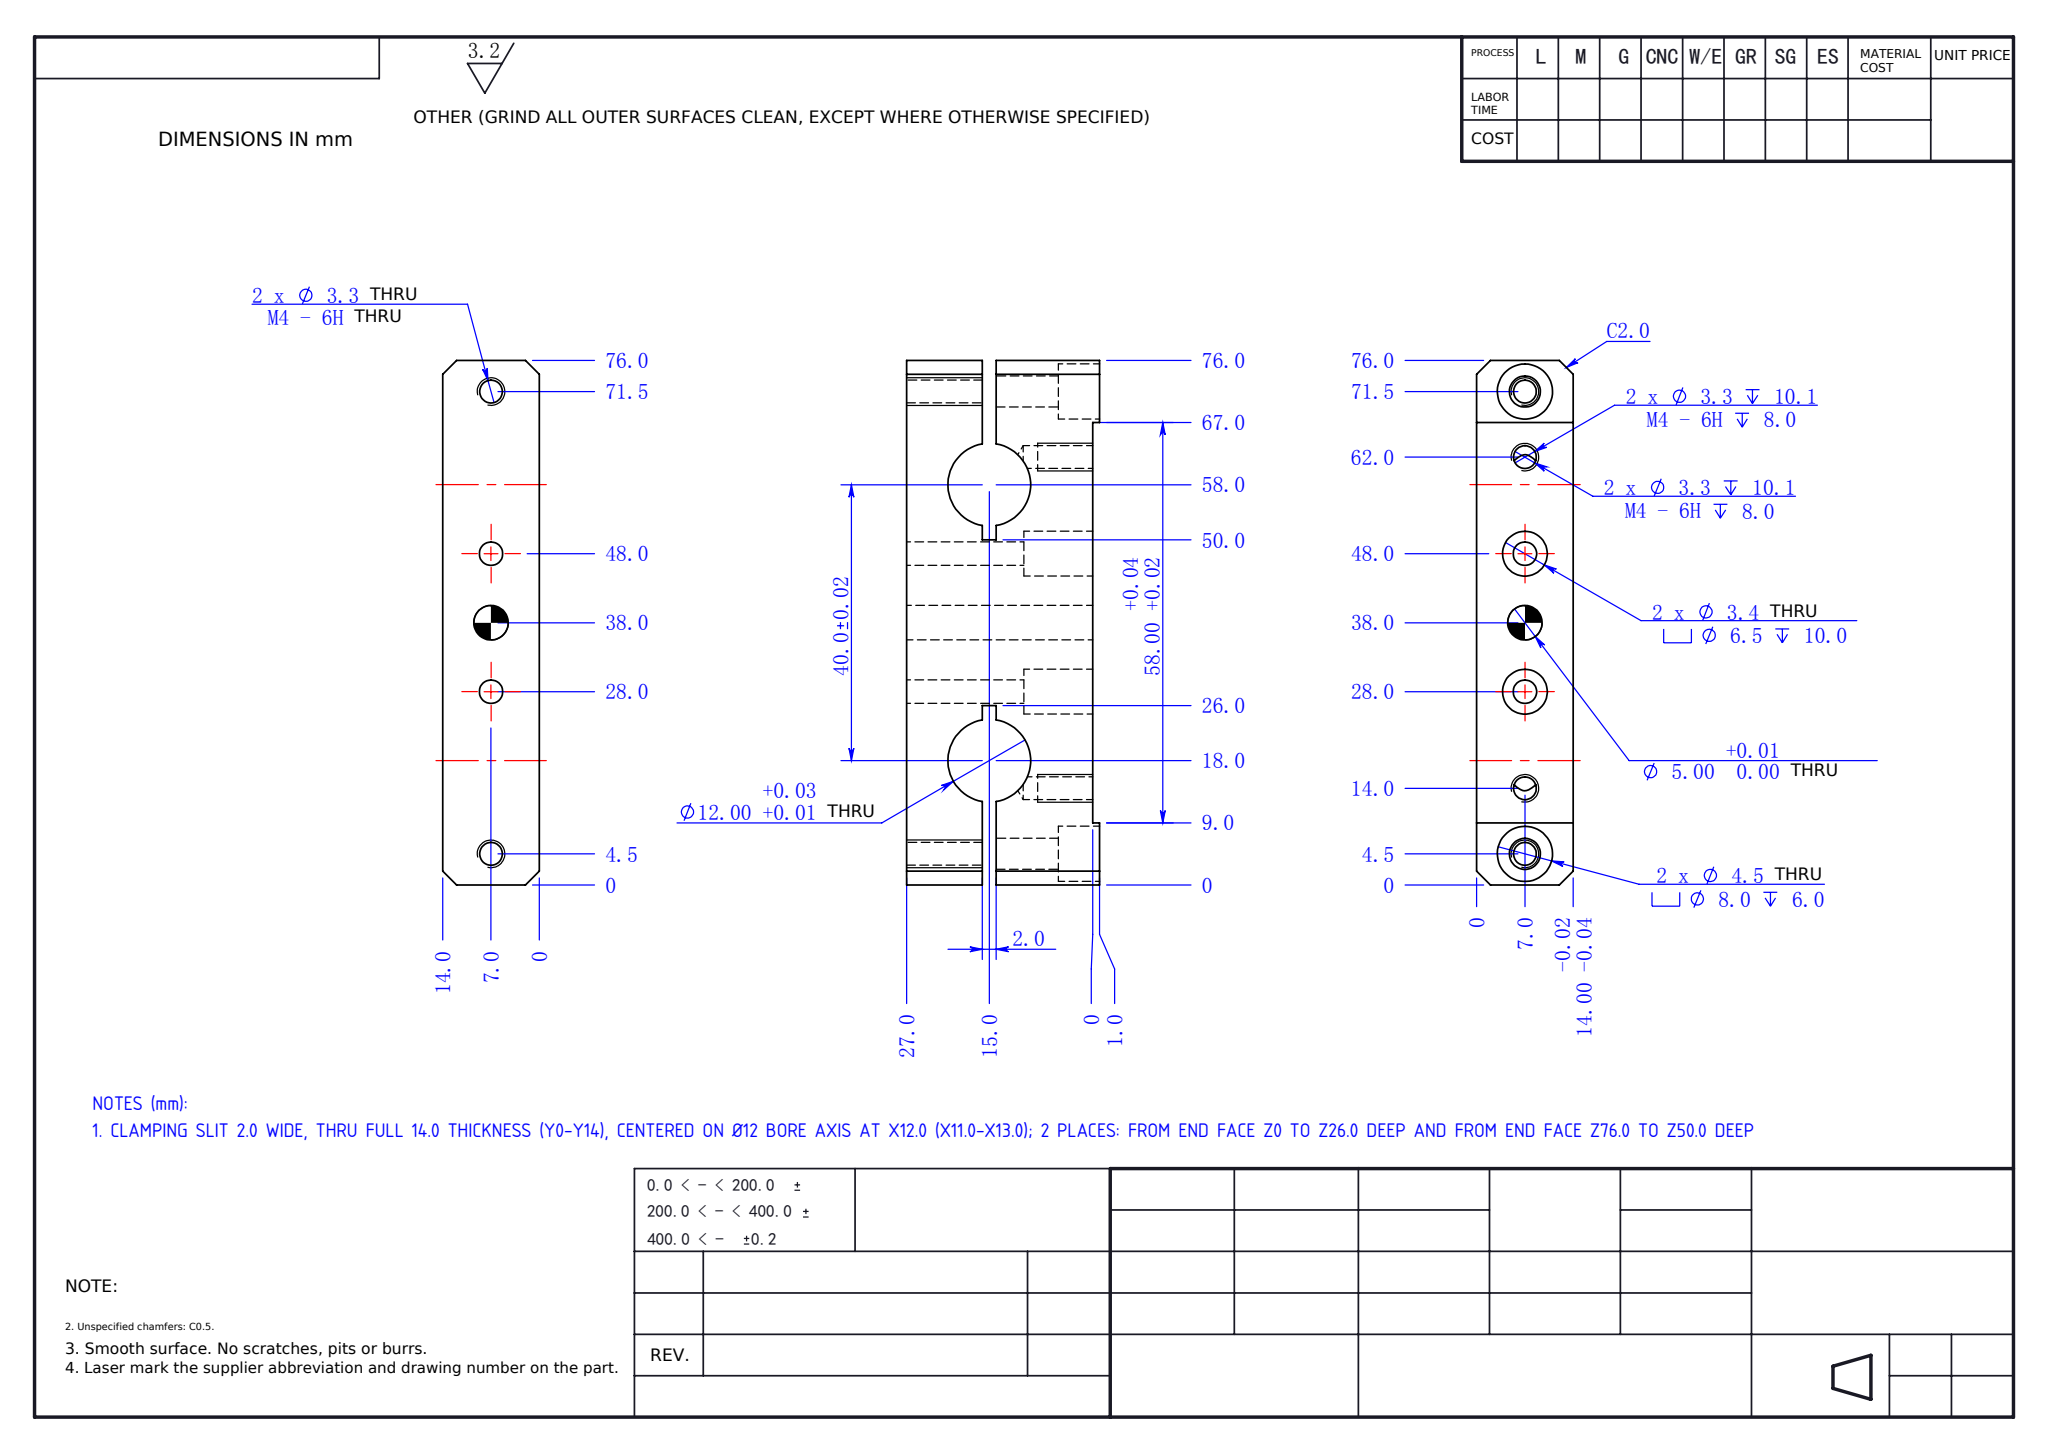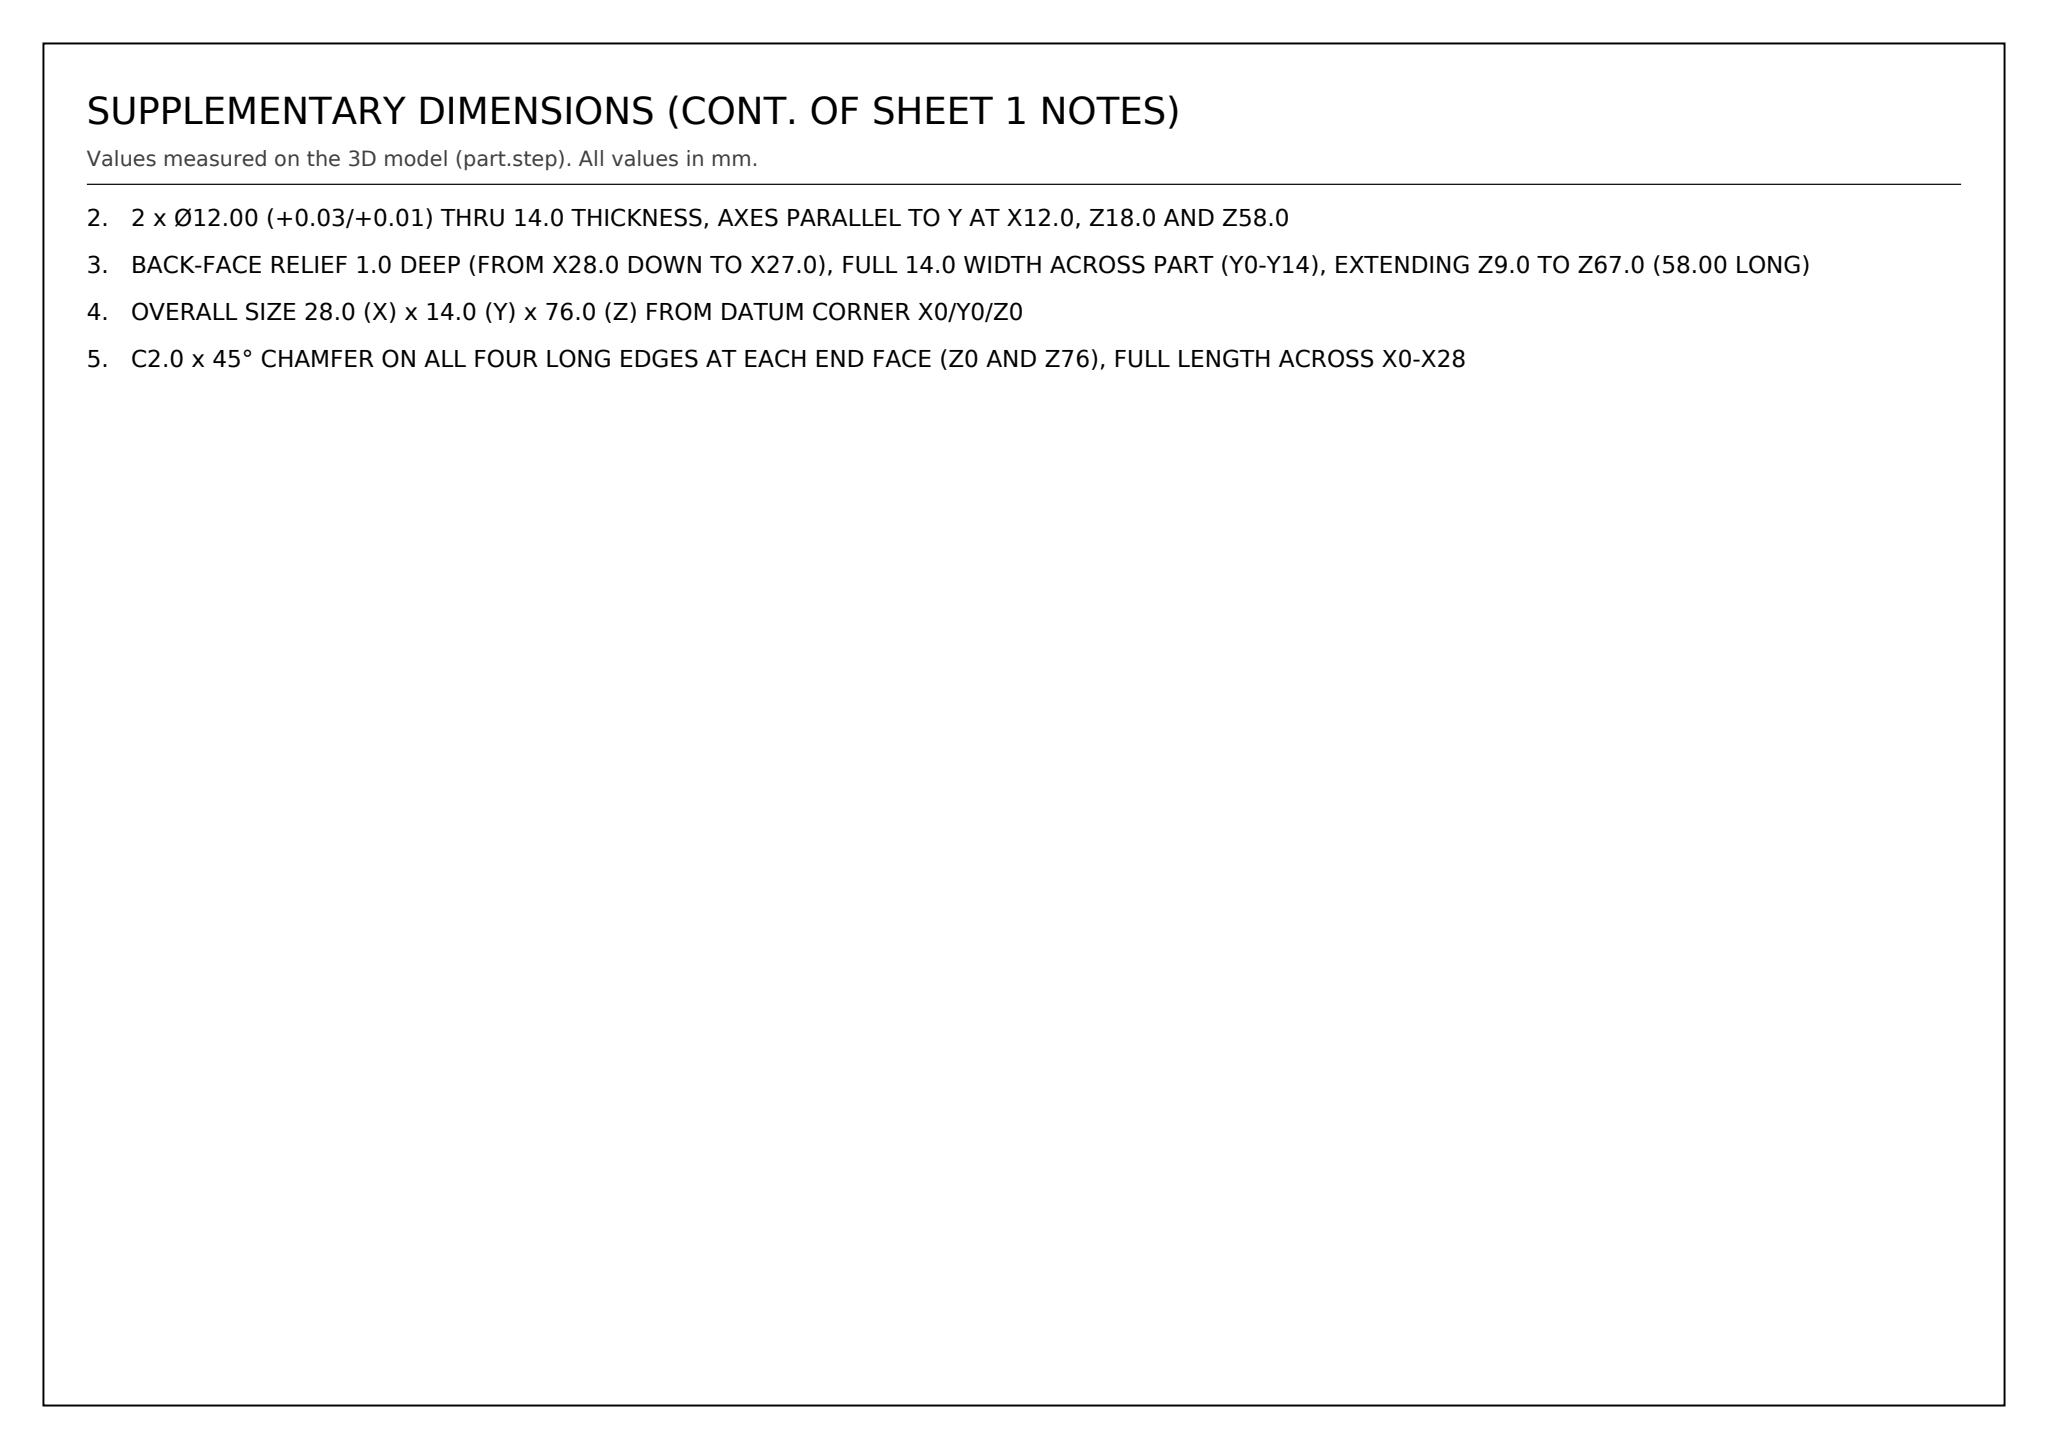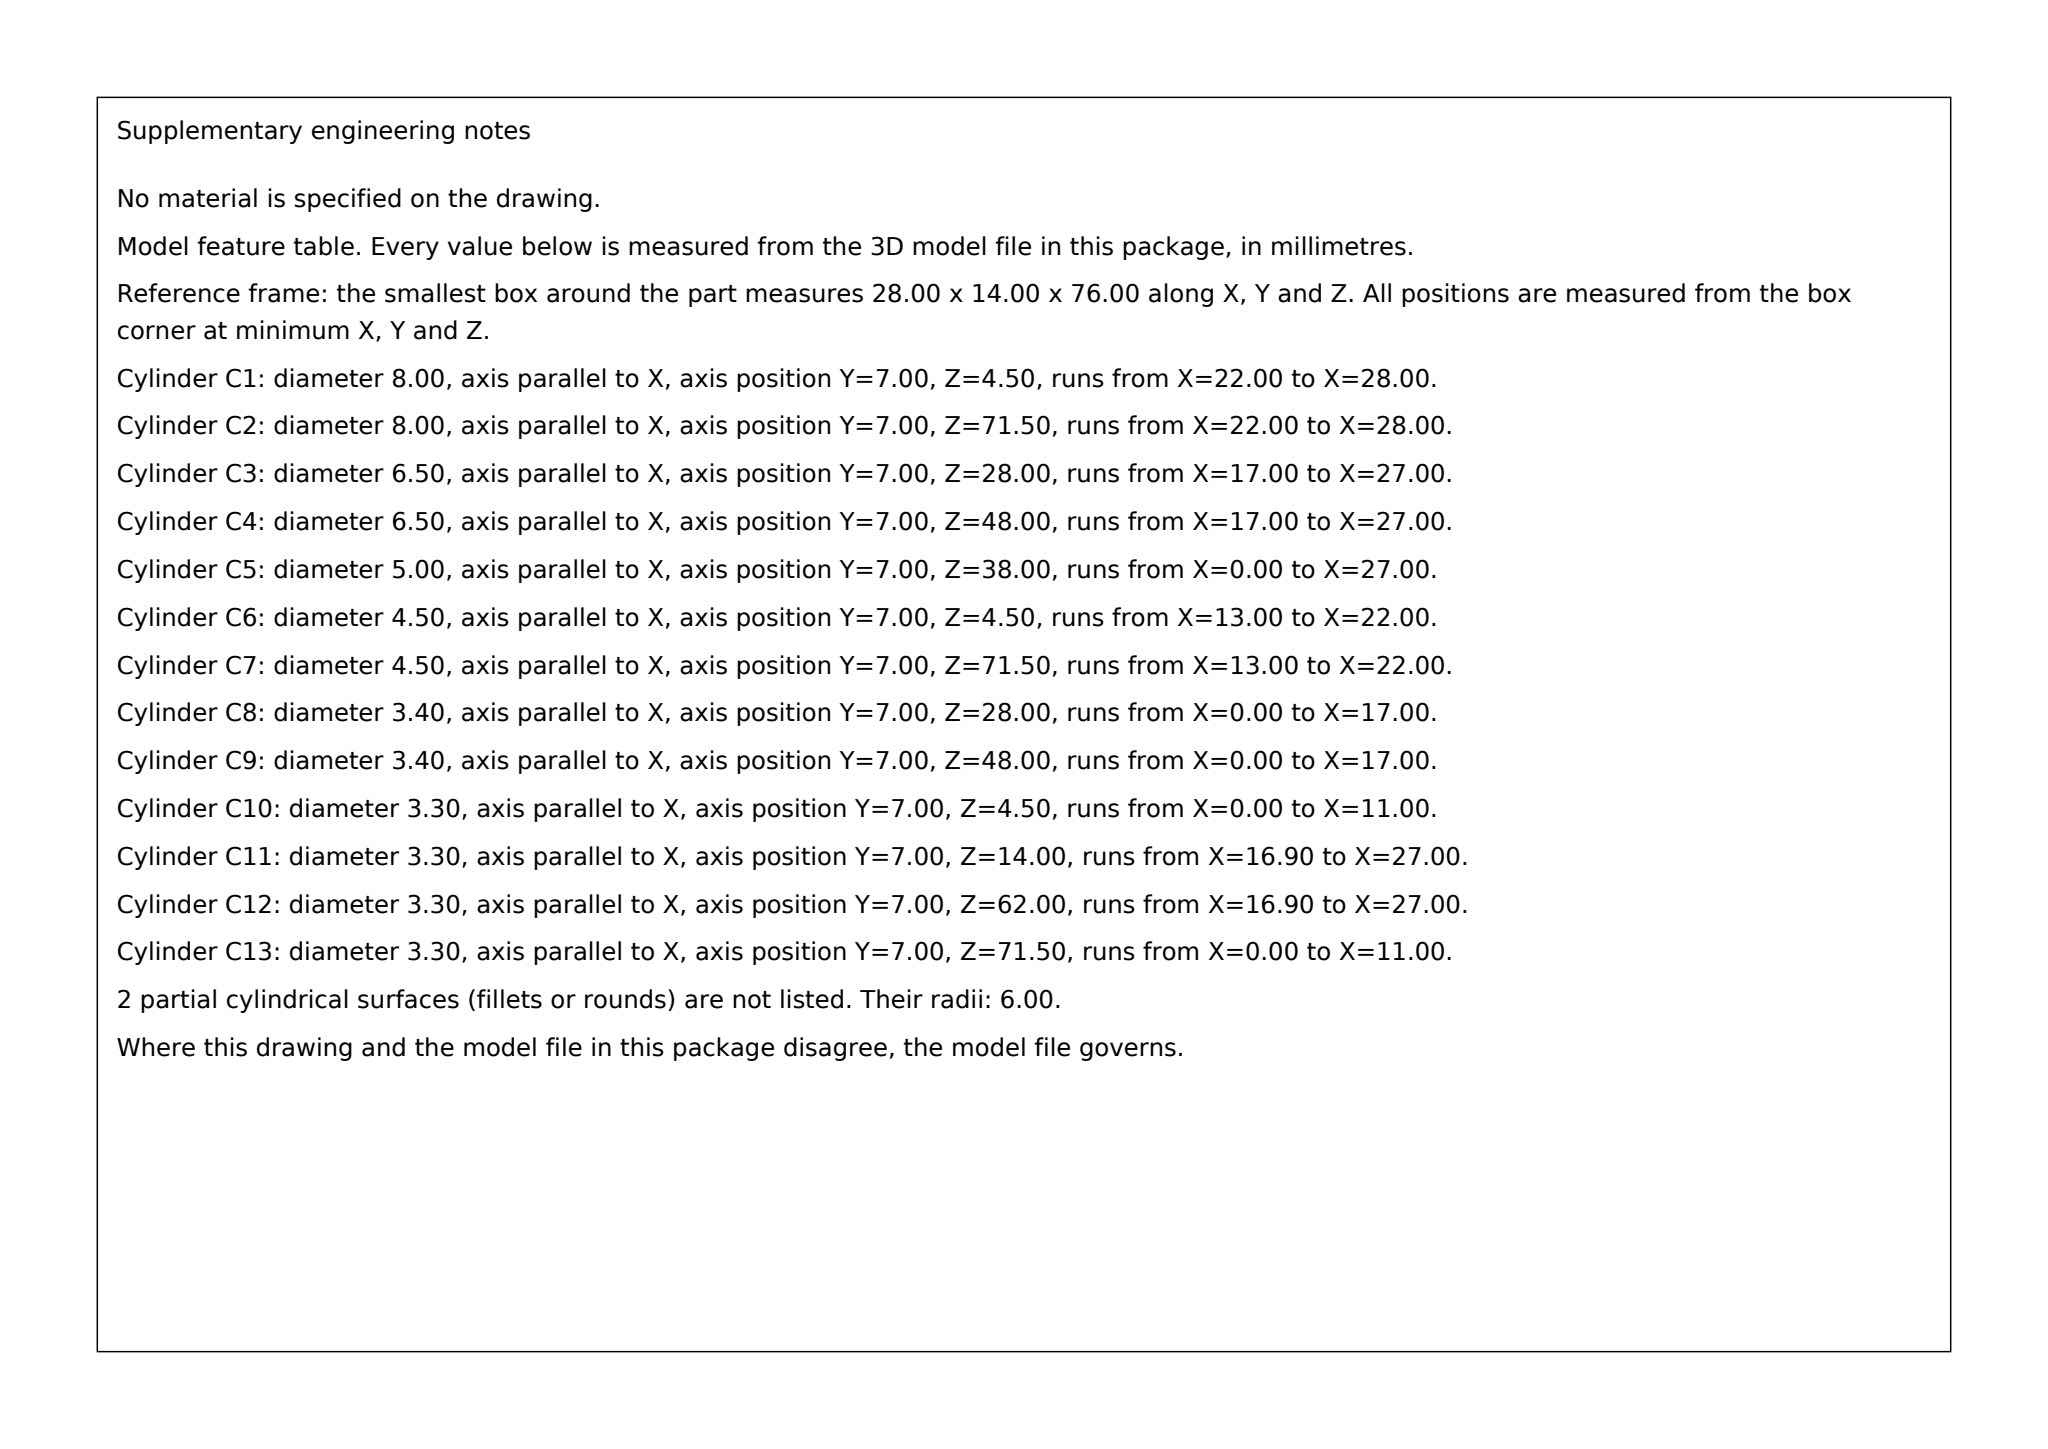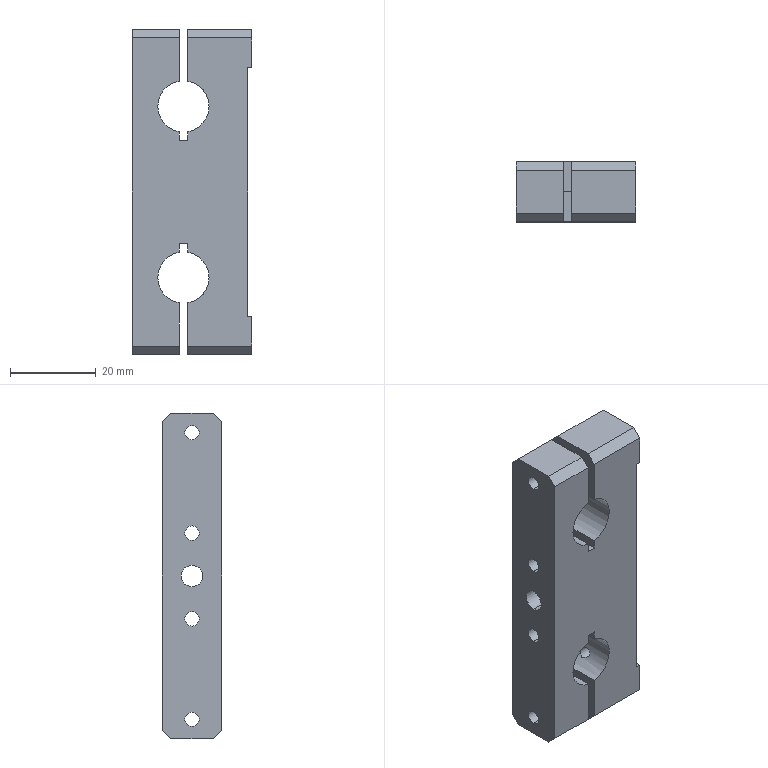Part | SolidWorks | mm | 1 solid | 67 faces | box 28 x 14 x 76 mm | volume 22063 mm3 | plane 34 | cylinder 30 | cone 3 | commonest cylinder face diameters 3.3 x8 8 x4 4.5 x4 6.5 x4 3.4 x4 12 x4 5 x2
Drawing notes:
CLAMPING SLIT 2.0 WIDE, THRU FULL 14.0 THICKNESS (Y0-Y14), CENTERED ON Ø12 BORE AXIS AT X12.0 (X11.0-X13.0); 2 PLACES: FROM END FACE Z0 TO Z26.0 DEEP AND FROM END FACE Z76.0 TO Z50.0 DEEP | from the solid: axis_planes x=11.0 and x=13.0, y extent [0,14], z extents [0,12.1],[23.9,26.0],[50.0,52.1],[63.9,76.0]; end planes z=26.0 and z=50.0 over x [11,13]
2 x Ø12.00 (+0.03/+0.01) THRU 14.0 THICKNESS, AXES PARALLEL TO Y AT X12.0, Z18.0 AND Z58.0 | from the solid: cylinders: two 12.0 dia arcs, axis y, positions [12.0,-,18.0] and [12.0,-,58.0], from y0 to y14
BACK-FACE RELIEF 1.0 DEEP (FROM X28.0 DOWN TO X27.0), FULL 14.0 WIDTH ACROSS PART (Y0-Y14), EXTENDING Z9.0 TO Z67.0 (58.00 LONG) | from the solid: axis_planes x=27.0 extent y[0,14] z[9,67]; x=28.0 extents z[0,9] and z[67,76]; z=9.0 and z=67.0 planes over x[27,28]
OVERALL SIZE 28.0 (X) x 14.0 (Y) x 76.0 (Z) FROM DATUM CORNER X0/Y0/Z0 | from the solid: bbox_xyz [28.0, 14.0, 76.0]
C2.0 x 45° CHAMFER ON ALL FOUR LONG EDGES AT EACH END FACE (Z0 AND Z76), FULL LENGTH ACROSS X0-X28 | from the solid: inclined_planes: eight 45° faces, size [11.0 or 15.0, 2.0, 2.0] at z=0 and z=74 origins, y=0 and y=12
build123d program:
from build123d import *

# Parameters (mm, degrees)
SKETCH1_W                                       = 28
SKETCH1_H                                       = 70
BOSS_EXTRUDE1_DEPTH                             = 7
SKETCH2_R                                       = 6
CUT_EXTRUDE1_DEPTH                              = 41.212
SKETCH3_W                                       = 2
SKETCH3_H                                       = 23
CUT_EXTRUDE2_DEPTH                              = 41.212
SKETCH8_W                                       = 1
SKETCH8_H                                       = 58
CUT_EXTRUDE5_DEPTH                              = 41.212
M4_TAPPED_HOLE2_D                               = 3.3
M4_TAPPED_HOLE2_DEPTH                           = 10.1
M4_TAPPED_HOLE2_TIP                             = 0.9914
M3_HEX_SOCKET_HEAD_CAP_SCREW_CBORE1_D           = 3.4
M3_HEX_SOCKET_HEAD_CAP_SCREW_CBORE1_CBORE_D     = 6.5
M3_HEX_SOCKET_HEAD_CAP_SCREW_CBORE1_CBORE_DEPTH = 10
SIZE_MM_DOWEL_PIN_HOLE_1_D                      = 5
SKETCH15_W                                      = 15
SKETCH15_H                                      = 14
SKETCH15_W_2                                    = 11
BOSS_EXTRUDE2_DEPTH                             = 3
SKETCH19_W                                      = 15
SKETCH19_H                                      = 14
SKETCH19_W_2                                    = 11
BOSS_EXTRUDE3_DEPTH                             = 3
M4_HEX_SOCKET_HEAD_CAP_SCREW_CBORE1_D           = 4.5
M4_HEX_SOCKET_HEAD_CAP_SCREW_CBORE1_DEPTH       = 15
M4_HEX_SOCKET_HEAD_CAP_SCREW_CBORE1_CBORE_D     = 8
M4_HEX_SOCKET_HEAD_CAP_SCREW_CBORE1_CBORE_DEPTH = 6
M4_TAPPED_HOLE3_D                               = 3.3
CHAMFER3_SIZE                                   = 2


with BuildPart() as part:
    # Sketch1 → Boss-Extrude1 (new, symmetric)
    with BuildSketch(Plane(origin=(0, 0, 0), x_dir=(1, 0, 0), z_dir=(0, 1, 0))):
        Rectangle(SKETCH1_W, SKETCH1_H)
    extrude(amount=BOSS_EXTRUDE1_DEPTH, both=True)

    # Sketch2 → Cut-Extrude1 (cut, through all)
    with BuildSketch(Plane(origin=(0, 7, 0), x_dir=(1, 0, 0), z_dir=(0, 1, 0))):
        with Locations(Location((-2, 20, 0), (0, 0, 270))):
            Circle(SKETCH2_R)
        with Locations(Location((-2, -20, 0), (0, 0, 90))):
            Circle(SKETCH2_R)
    extrude(amount=-CUT_EXTRUDE1_DEPTH, mode=Mode.SUBTRACT)

    # Sketch3 → Cut-Extrude2 (cut, through all)
    with BuildSketch(Plane(origin=(0, 7, 0), x_dir=(1, 0, 0), z_dir=(0, 1, 0))):
        with Locations((-2, 23.5)):
            Rectangle(SKETCH3_W, SKETCH3_H)
        with Locations((-2, -23.5)):
            Rectangle(SKETCH3_W, SKETCH3_H)
    extrude(amount=-CUT_EXTRUDE2_DEPTH, mode=Mode.SUBTRACT)

    # Sketch8 → Cut-Extrude5 (cut, through all)
    with BuildSketch(Plane(origin=(0, 7, 0), x_dir=(1, 0, 0), z_dir=(0, 1, 0))):
        with Locations((13.5, 0)):
            Rectangle(SKETCH8_W, SKETCH8_H)
    extrude(amount=-CUT_EXTRUDE5_DEPTH, mode=Mode.SUBTRACT)

    # M4 Tapped Hole2
    with Locations(Plane(origin=(13, 0, 0), x_dir=(0, 0, -1), z_dir=(1, 0, 0))):
        with Locations((-24, 0), (24, 0)):
            Hole(M4_TAPPED_HOLE2_D / 2, depth=M4_TAPPED_HOLE2_DEPTH)
            with Locations((0, 0, -(M4_TAPPED_HOLE2_DEPTH + M4_TAPPED_HOLE2_TIP / 2))):  # 118° drill point
                Cone(0, M4_TAPPED_HOLE2_D / 2, M4_TAPPED_HOLE2_TIP, mode=Mode.SUBTRACT)

    # M3 Hex Socket Head Cap Screw CBORE1 (through all)
    with Locations(Plane(origin=(13, 0, 0), x_dir=(0, 0, -1), z_dir=(1, 0, 0))):
        with Locations((-10, 0), (10, 0)):
            CounterBoreHole(M3_HEX_SOCKET_HEAD_CAP_SCREW_CBORE1_D / 2, M3_HEX_SOCKET_HEAD_CAP_SCREW_CBORE1_CBORE_D / 2, M3_HEX_SOCKET_HEAD_CAP_SCREW_CBORE1_CBORE_DEPTH)

    # Size mm Dowel Pin Hole 1 (through all)
    with Locations(Plane(origin=(13, 0, 0), x_dir=(0, 0, -1), z_dir=(1, 0, 0))):
        with Locations((0, 0)):
            Hole(SIZE_MM_DOWEL_PIN_HOLE_1_D / 2)

    # Sketch15 → Boss-Extrude2 (add)
    with BuildSketch(Plane(origin=(0, 0, -35), x_dir=(-1, 0, 0), z_dir=(0, 0, -1))):
        with Locations((-6.5, 0)):
            Rectangle(SKETCH15_W, SKETCH15_H)
        with Locations((8.5, 0)):
            Rectangle(SKETCH15_W_2, SKETCH15_H)
    extrude(amount=BOSS_EXTRUDE2_DEPTH)

    # Sketch19 → Boss-Extrude3 (add)
    with BuildSketch(Plane.XY.offset(35)):
        with Locations((6.5, 0)):
            Rectangle(SKETCH19_W, SKETCH19_H)
        with Locations((-8.5, 0)):
            Rectangle(SKETCH19_W_2, SKETCH19_H)
    extrude(amount=BOSS_EXTRUDE3_DEPTH)

    # M4 Hex Socket Head Cap Screw CBORE1
    with Locations(Plane(origin=(14, 0, 0), x_dir=(0, 0, -1), z_dir=(1, 0, 0))):
        with Locations((33.5, 0), (-33.5, 0)):
            CounterBoreHole(M4_HEX_SOCKET_HEAD_CAP_SCREW_CBORE1_D / 2, M4_HEX_SOCKET_HEAD_CAP_SCREW_CBORE1_CBORE_D / 2, M4_HEX_SOCKET_HEAD_CAP_SCREW_CBORE1_CBORE_DEPTH, depth=M4_HEX_SOCKET_HEAD_CAP_SCREW_CBORE1_DEPTH)

    # M4 Tapped Hole3 (through all)
    with Locations(Plane(origin=(-3, 0, 0), x_dir=(0, 0, -1), z_dir=(1, 0, 0))):
        with Locations((-33.5, 0), (33.5, 0)):
            Hole(M4_TAPPED_HOLE3_D / 2)

    # Chamfer3
    chamfer3_edges = [part.edges().sort_by_distance(p)[0] for p in [
        (6.5, -7, -38),
        (6.5, 7, -38),
        (-8.5, 7, -38),
        (-8.5, -7, -38),
        (6.5, 7, 38),
        (6.5, -7, 38),
        (-8.5, -7, 38),
        (-8.5, 7, 38),
    ]]
    chamfer(chamfer3_edges, length=CHAMFER3_SIZE)


solid = part.part